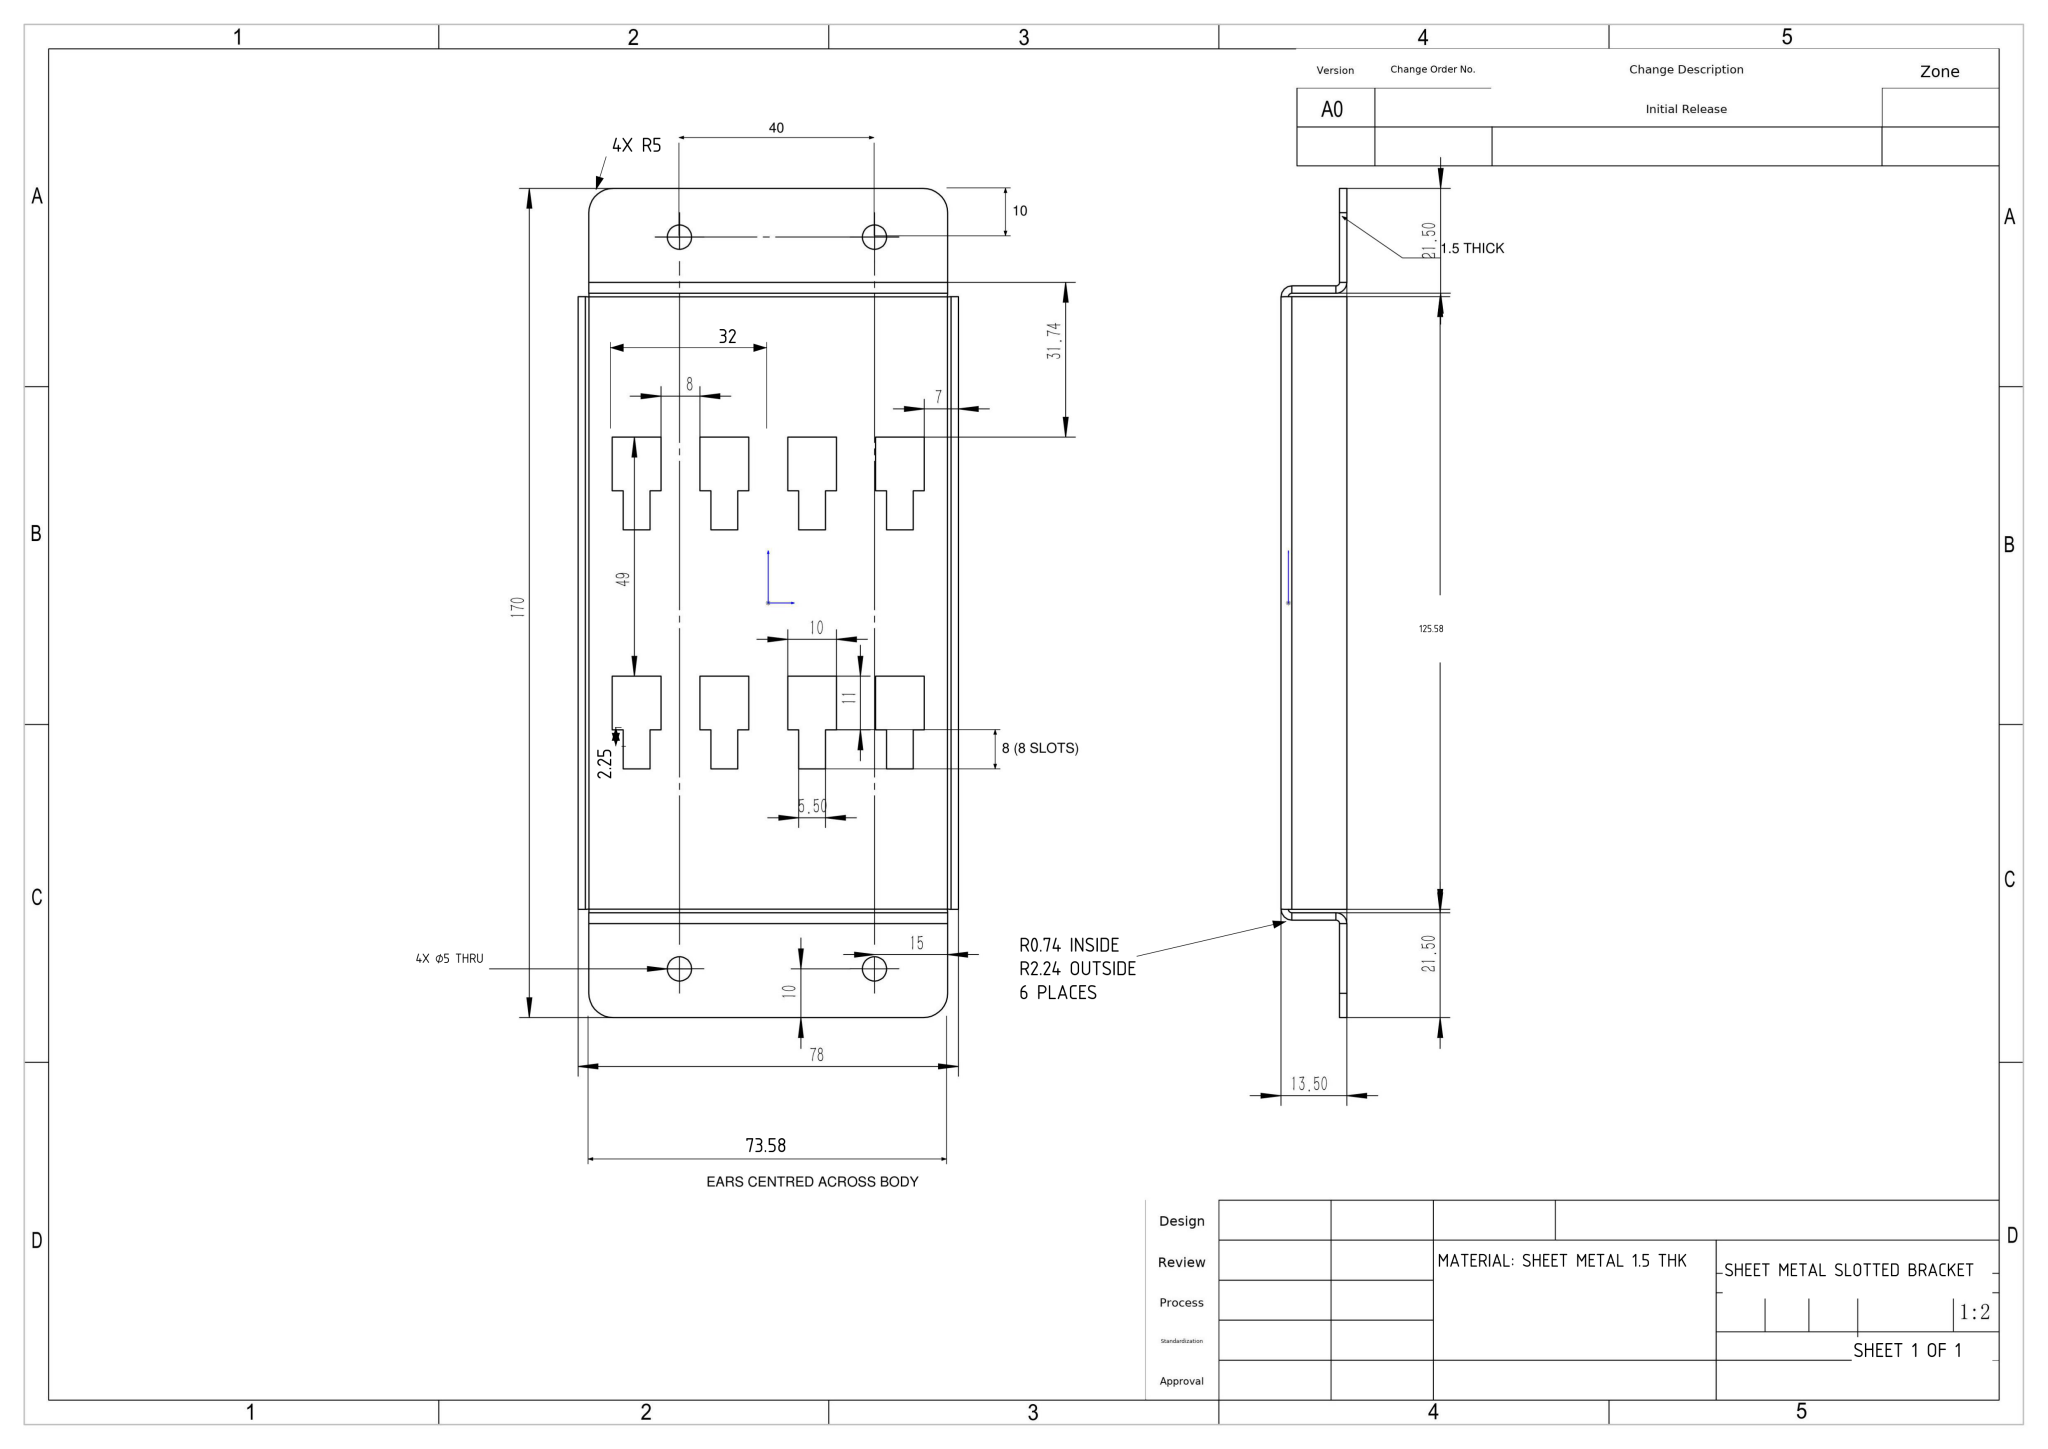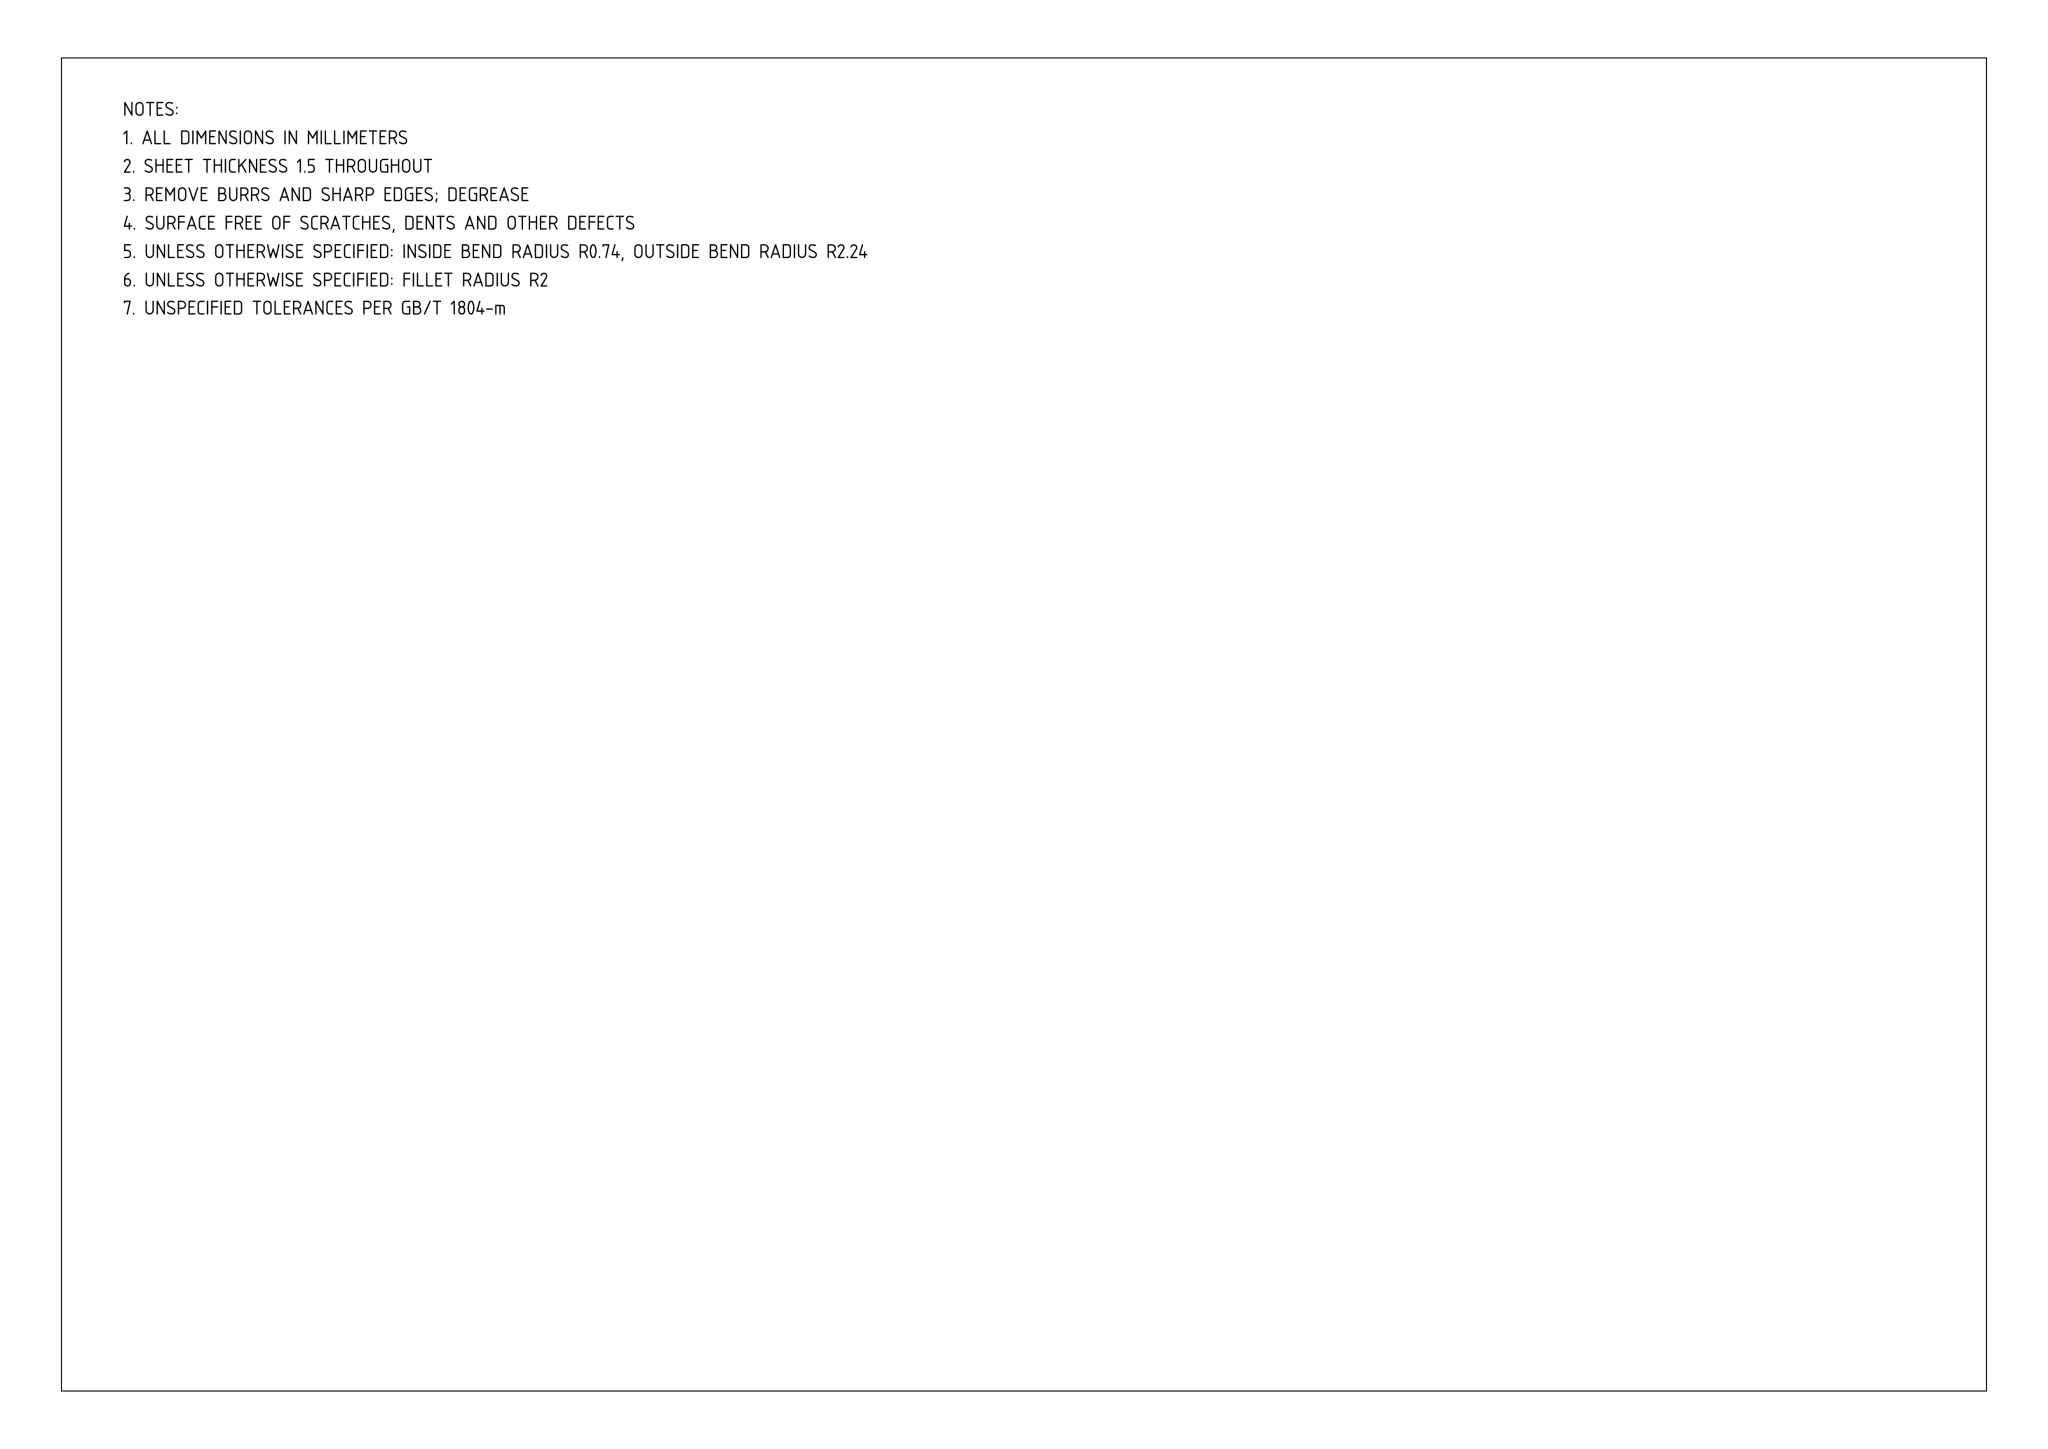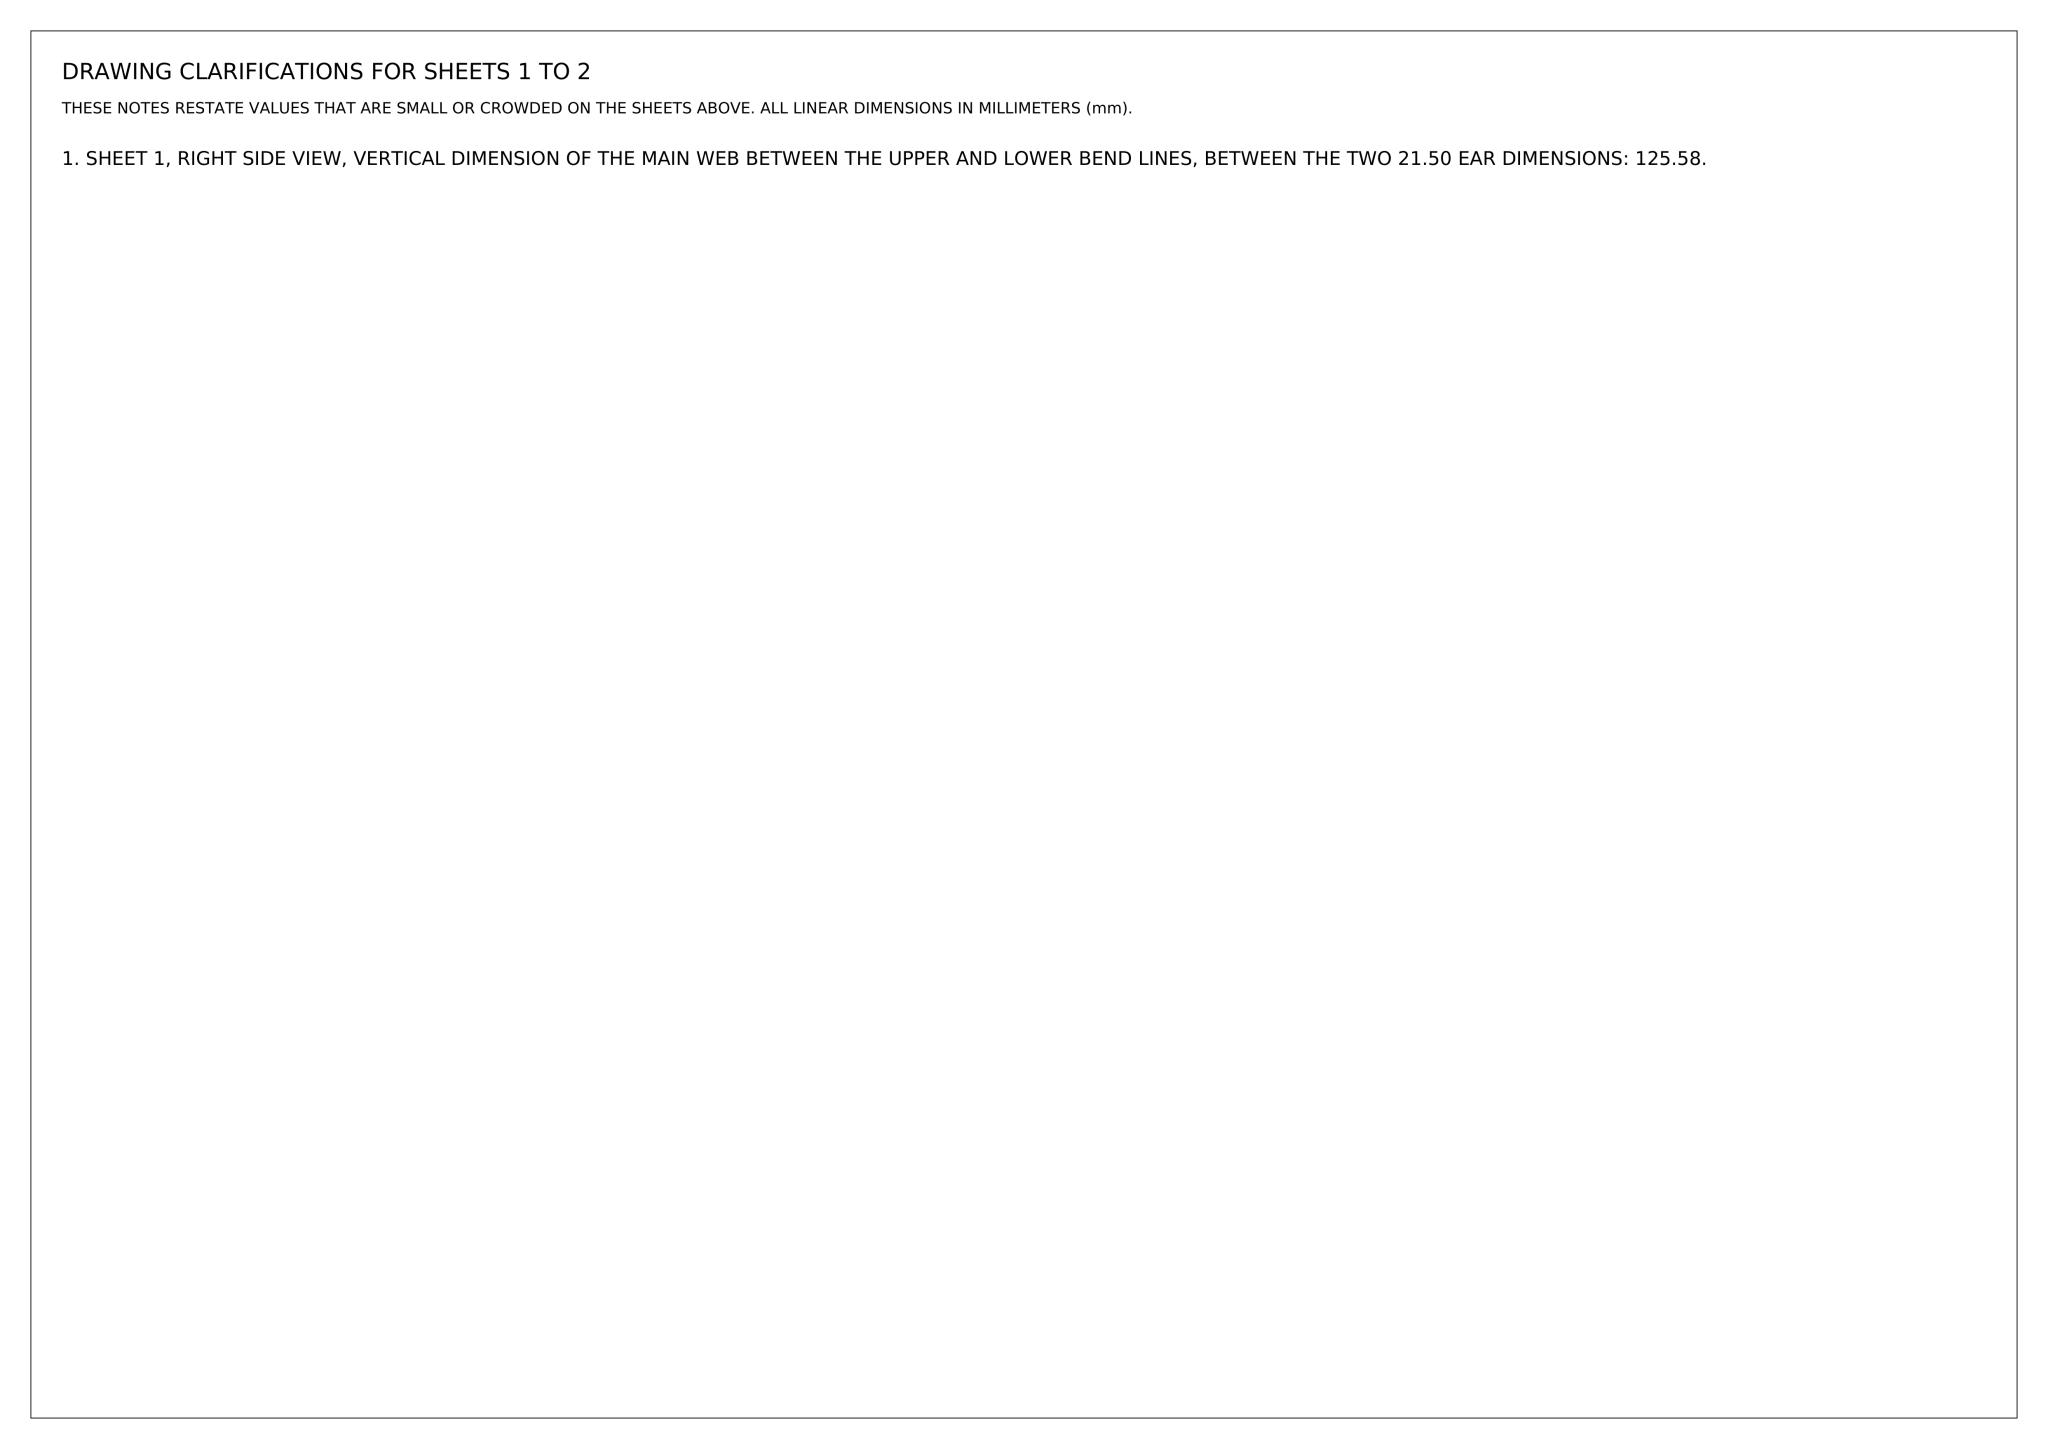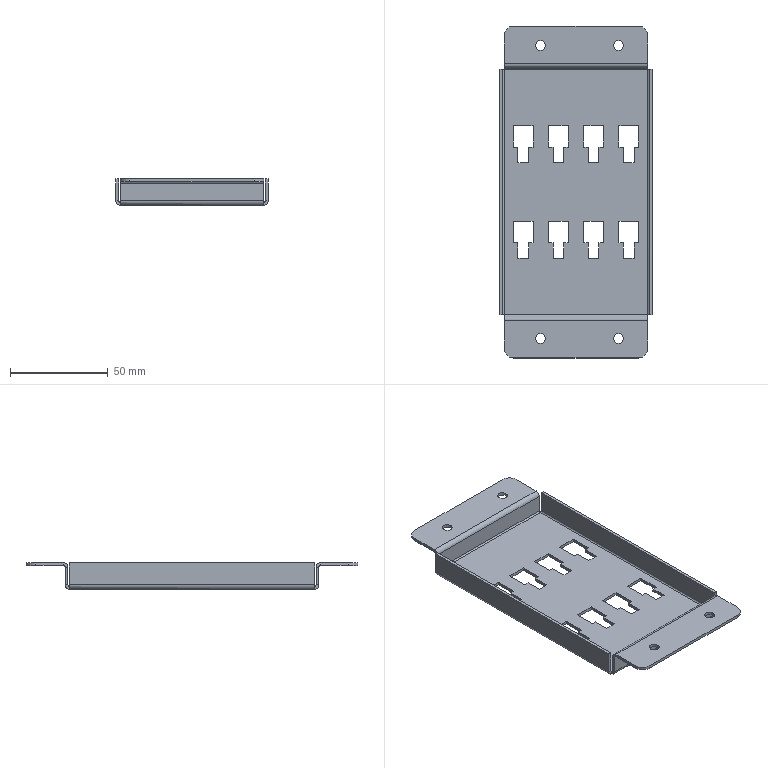Part | NX | mm | 1 solid | 130 faces | box 78 x 170 x 13.5 mm | volume 24246 mm3 | plane 98 | cylinder 24 | spline 8 | commonest cylinder face diameters 5 x8 4.473 x6 1.473 x6 10 x4